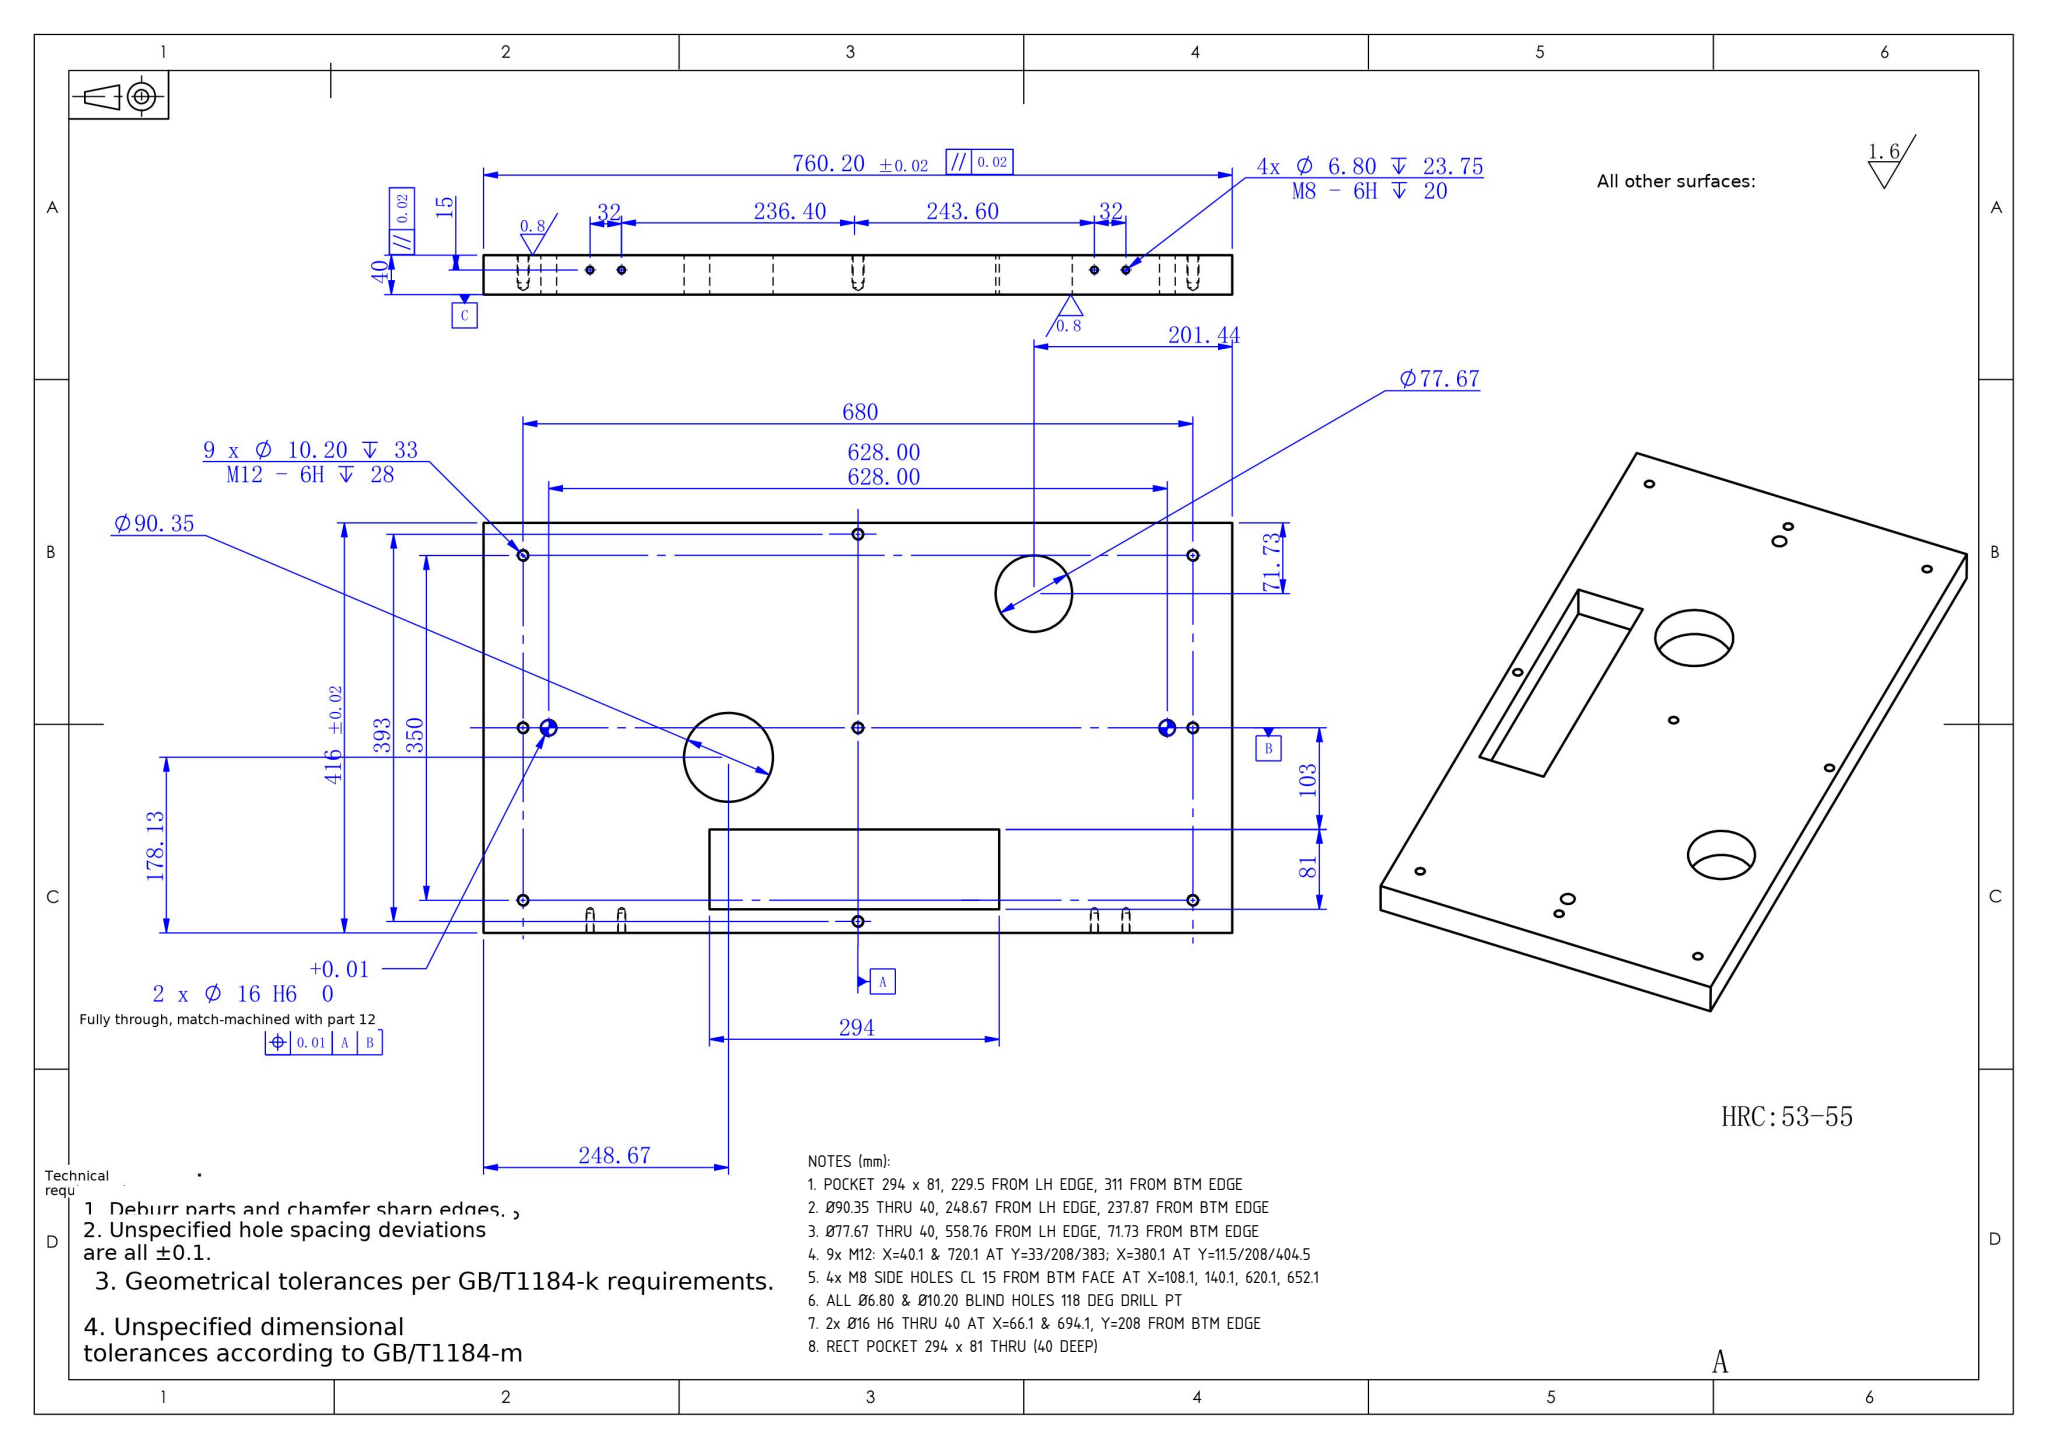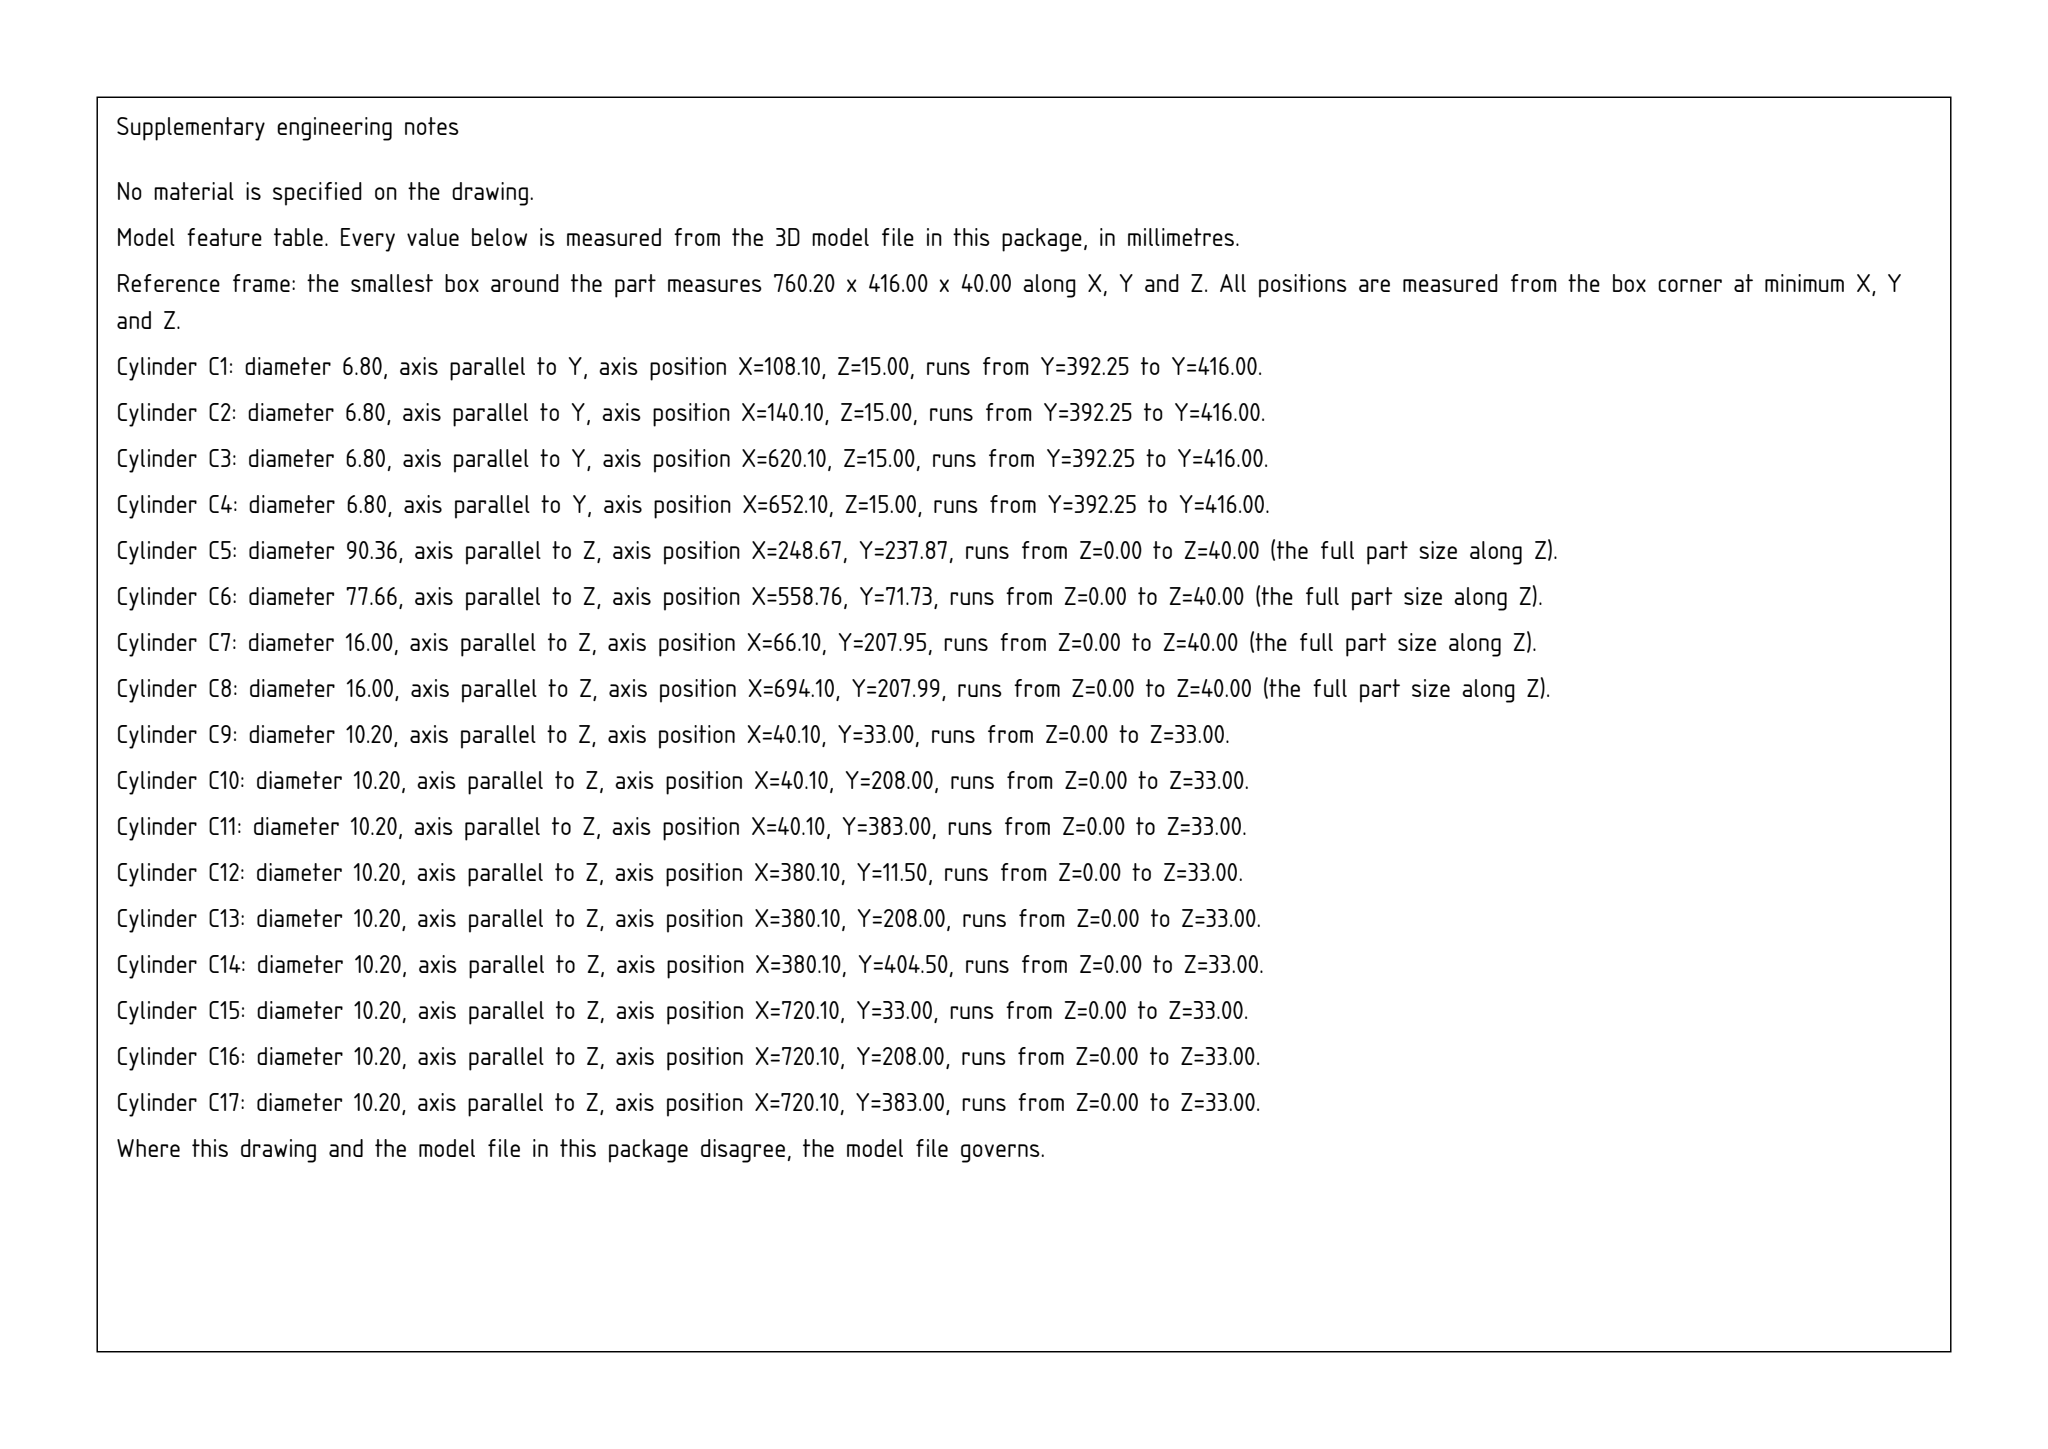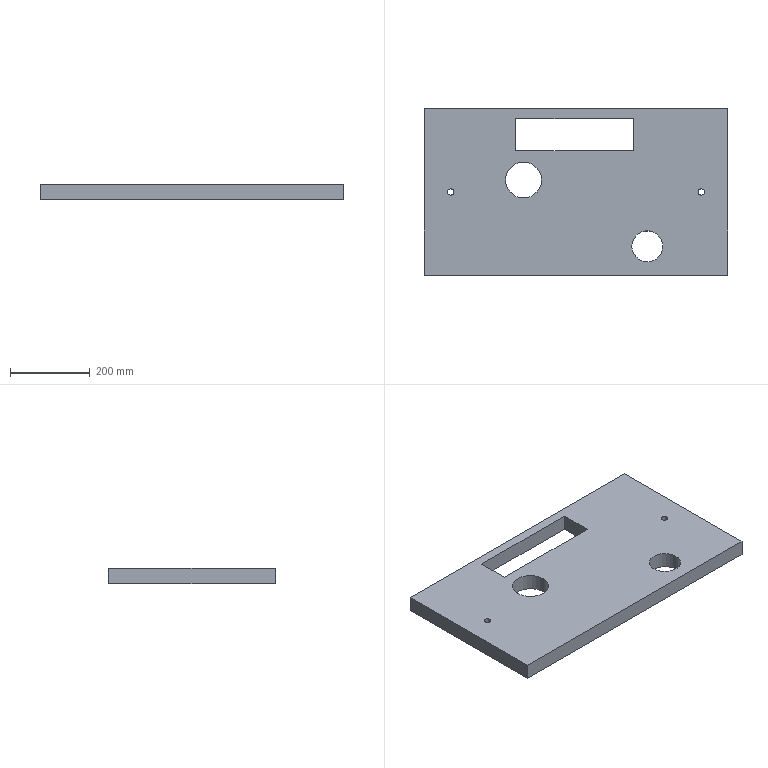Part | SolidWorks | mm | 1 solid | 70 faces | box 760.2 x 416 x 40 mm | volume 11206559 mm3 | cylinder 34 | cone 26 | plane 10 | commonest cylinder face diameters 10.2 x18 6.8 x8 16 x4 90.351 x2 77.665 x2
Drawing notes:
POCKET 294 x 81, 229.5 FROM LH EDGE, 311 FROM BTM EDGE | from the solid: axis planes x=229.5/523.5 (294 lg), y=311/392 (81 wd)
Ø90.35 THRU 40, 248.67 FROM LH EDGE, 237.87 FROM BTM EDGE | from the solid: cyl dia 90.351 axis z at (248.67, 237.87), length 40 = plate thk
Ø77.67 THRU 40, 558.76 FROM LH EDGE, 71.73 FROM BTM EDGE | from the solid: cyl dia 77.665 axis z at (558.76, 71.73), length 40 = plate thk
9x M12: X=40.1 & 720.1 AT Y=33/208/383; X=380.1 AT Y=11.5/208/404.5 | from the solid: 10.2 dia z-holes at (40.1/720.1, 33/208/383) and (380.1, 11.5/208/404.5)
4x M8 SIDE HOLES CL 15 FROM BTM FACE AT X=108.1, 140.1, 620.1, 652.1 | from the solid: 6.8 dia y-axis cyls at z=15, x=108.1/140.1/620.1/652.1, lg 23.75
ALL Ø6.80 & Ø10.20 BLIND HOLES 118 DEG DRILL PT | from the solid: cones 118 deg on ref dia 6.8 (8x) and 10.2 (18x)
2x Ø16 H6 THRU 40 AT X=66.1 & 694.1, Y=208 FROM BTM EDGE | from the solid: 16.0 dia z-cyls at (66.1,207.95) and (694.1,208), length 40
RECT POCKET 294 x 81 THRU (40 DEEP) | from the solid: Planes x=229.5/523.5 (294) and y=311/392 (81); only z-planes at 0 and 40, no pocket floor -> pocket passes through 40 thk
build123d program:
from build123d import *

# Parameters (mm, degrees)
SKETCH1_W                  = 760.2
SKETCH1_H                  = 416
BOSS_EXTRUDE1_DEPTH        = 40
M12_TAPPED_HOLE1_D         = 10.2
M12_TAPPED_HOLE1_DEPTH     = 33
M12_TAPPED_HOLE1_TIP       = 3.064
M8_TAPPED_HOLE1_AT_2_COUNT = 2
M8_TAPPED_HOLE1_AT_2_PITCH = 32
F_16_0_16_DIAMETER_HOLE1_D = 16
SKETCH14_W                 = 294
SKETCH14_H                 = 81
CUT_EXTRUDE2_DEPTH         = 746.409
SKETCH15_R                 = 45.176
SKETCH15_R_2               = 38.833
CUT_EXTRUDE3_DEPTH         = 80


with BuildPart() as part:
    # Sketch1 → Boss-Extrude1 (new body)
    with BuildSketch(Plane.XY):
        with Locations((272.129, -150.652)):
            Rectangle(SKETCH1_W, SKETCH1_H)
    extrude(amount=BOSS_EXTRUDE1_DEPTH)

    # M12 Tapped Hole1
    with Locations(Plane(origin=(0, 0, 0), x_dir=(-1, 0, 0), z_dir=(0, 0, -1))):
        with Locations((-612.129, -325.652), (-612.129, -150.652), (-612.129, 24.348), (-272.129, 45.848), (-272.129, -150.652), (-272.129, -347.152), (67.871, -325.652), (67.871, -150.652), (67.871, 24.348)):
            Hole(M12_TAPPED_HOLE1_D / 2, depth=M12_TAPPED_HOLE1_DEPTH)
            with Locations((0, 0, -(M12_TAPPED_HOLE1_DEPTH + M12_TAPPED_HOLE1_TIP / 2))):  # 118° drill point
                Cone(0, M12_TAPPED_HOLE1_D / 2, M12_TAPPED_HOLE1_TIP, mode=Mode.SUBTRACT)

    # Sketch7 → M8 Tapped Hole1 (revolve, cut)
    with BuildSketch(Plane(origin=(0.1293, 57.348, 15), x_dir=(0, 0, 1), z_dir=(1, 0, 0))):
        Polygon((0, 0), (0, 25.793), (3.4, 23.75), (3.4, 0), align=None)
    m8_tapped_hole1 = revolve(axis=Axis((0.1293, 63.698, 15), (0, -1, 0)), mode=Mode.SUBTRACT)

    # M8 Tapped Hole1 at 2: M8 Tapped Hole1 ×2
    with Locations(*[(i * M8_TAPPED_HOLE1_AT_2_PITCH, 0, 0) for i in range(1, M8_TAPPED_HOLE1_AT_2_COUNT)]):
        add(m8_tapped_hole1, mode=Mode.SUBTRACT)

    # Mirror3: M8 Tapped Hole1 across plane
    add(m8_tapped_hole1.mirror(Plane(origin=(272.129, 0, 0), x_dir=(0, 0, 1), z_dir=(1, 0, 0))), mode=Mode.SUBTRACT)

    # Mirror3 copy 1 sketch → Mirror3 copy 1 (revolve, cut)
    with BuildSketch(Plane(origin=(512.129, 57.348, 15), x_dir=(0, 0, 1), z_dir=(-1, 0, 0))):
        Polygon((0, 0), (0, -25.793), (3.4, -23.75), (3.4, 0), align=None)
    revolve(axis=Axis((512.129, 63.698, 15), (0, 1, 0)), mode=Mode.SUBTRACT)

    # 16.0 _16_ Diameter Hole1 (through all)
    with Locations(Plane(origin=(0, 0, 0), x_dir=(-1, 0, 0), z_dir=(0, 0, -1))):
        with Locations((41.871, -150.697), (-586.129, -150.656)):
            Hole(F_16_0_16_DIAMETER_HOLE1_D / 2)

    # Sketch14 → Cut-Extrude2 (cut, through all)
    with BuildSketch(Plane.XY.offset(40)):
        with Locations((268.529, -7.152)):
            Rectangle(SKETCH14_W, SKETCH14_H)
    extrude(amount=-CUT_EXTRUDE2_DEPTH, mode=Mode.SUBTRACT)

    # Sketch15 → Cut-Extrude3 (cut)
    with BuildSketch(Plane.XY.offset(40)):
        with Locations((140.695, -120.78)):
            Circle(SKETCH15_R)
        with Locations((450.788, -286.922)):
            Circle(SKETCH15_R_2)
    extrude(amount=-CUT_EXTRUDE3_DEPTH, mode=Mode.SUBTRACT)


solid = part.part